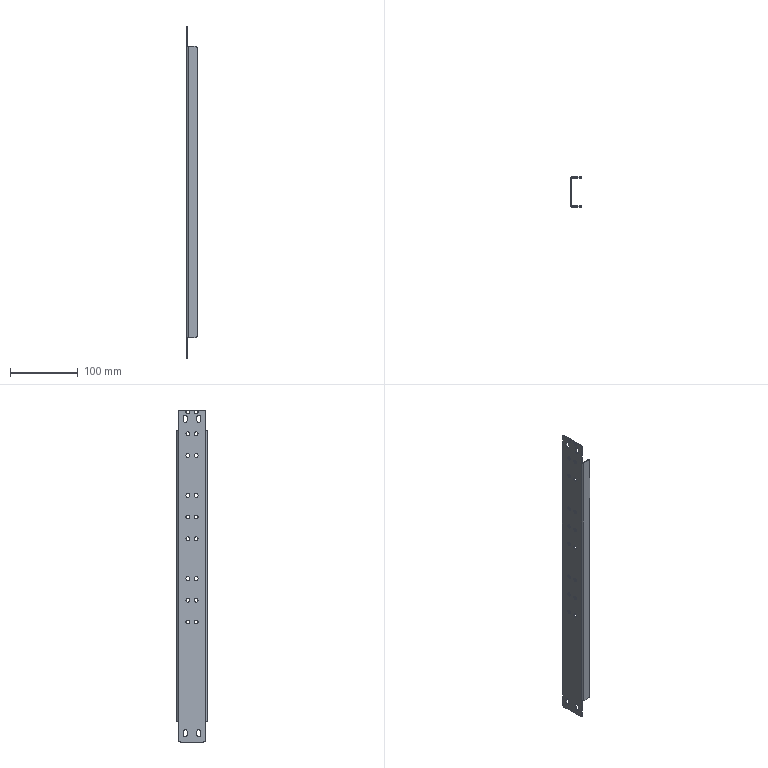Component | SolidWorks | FuseGroupMountingBeam100-9 | 1 solid | 90 faces | volume 47958 mm3 | cylinder 60 | plane 30 | commonest cylinder face diameters 5.5 x48 6 x8 4.473 x2 1.473 x2